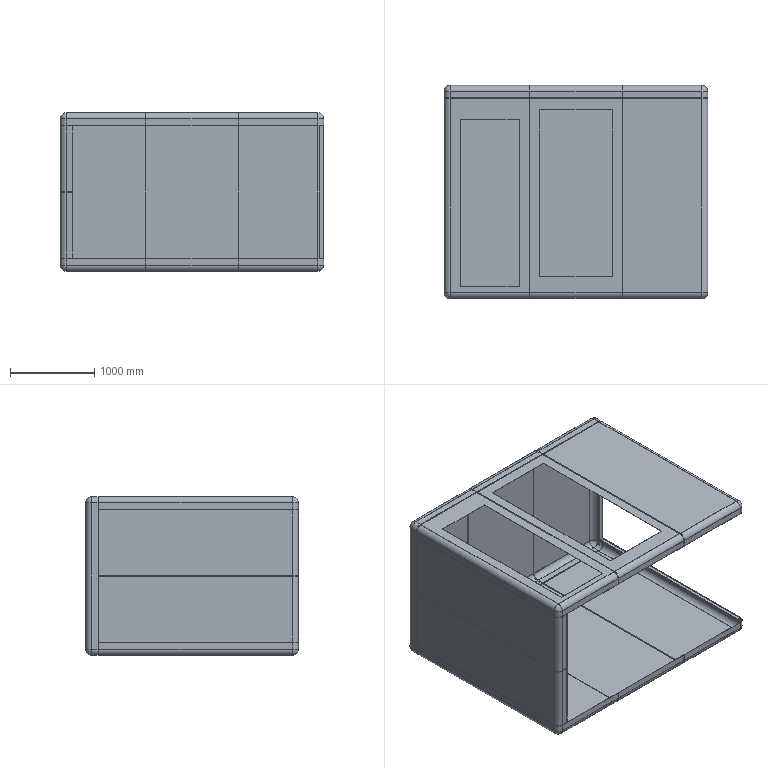Assembly | SolidWorks | mm | 23 component files | 23 solids | 472 faces | box 3131 x 2531 x 1881 mm | volume 75496655 mm3 | plane 358 | cylinder 98 | torus 16 | commonest cylinder face diameters 139 x35 133 x35 141 x8 135 x8 10 x6 4 x6
Bill of materials:
A-SideAluminumCasing1 | 1 |  | Thin rectangular frame-like plate with a large central rectangular opening; one long edge turns down with a rounded bend, forming a short flange.
A-SideAluminumCasing2 | 1 |  | Thin rectangular frame-like plate with a large central rectangular opening and one long edge rolled down into a short rounded flange.
A-SideAluminumCasing3 | 1 |  | Solid rectangular plate or shallow cover with no openings and rounded edges and corners on at least two adjacent sides.
A-SideSealant | 1 |  | Very thin, long sheet or strip; both ends appear turned through small rounded bends.
C-SideSealant1 | 7 |  | Very thin, long sheet or strip with a small rounded bend at one end only.
C-SideAluminumCasing1 | 1 |  | Flat rectangular sheet with one long edge bent down into a short flange with a small radius.
C-SideAluminumCasing2 | 1 |  | Rectangular sheet panel; one long edge is bent down and the opposite long edge appears turned up with a radius, giving an offset or stepped edge profile.
C-SideAluminumCasing3 | 1 |  | Rectangular tray-like sheet panel with a rounded downturned edge along one long side and short raised lips at the short ends.
C-SideSealant | 1 |  | Very thin, long sheet or strip with both ends turned through small rounded bends, apparently in the opposite direction to the similar strip parts.
D-SideAluminumCasing | 2 |  | Rectangular sheet panel standing on edge, with a short return flange formed by a small rounded bend along one edge (an L-like profile).
D-SideSealant | 1 |  | Flat thin rectangular sheet or plate with no visible holes, bends or edge features.
CasingA | 1 |  | Rectangular plate or panel of noticeable thickness with rounded edges and corners on several sides, giving a soft-edged slab shape.
CasingB | 1 |  | Thin-walled shallow channel (C-profile) with constant cross-section: a wide flat web with a short flange along each long edge, joined by radiused bends; both ends open.
CasingC | 1 |  | Thin-walled channel of similar C-profile to unnamed part, but closed at one end by an end wall with rounded corners, making a shallow tray-like cap; the other end is open.
Sealant | 2 |  | Very thin, narrow C-shaped profile element: a long straight segment with short angled/curved returns at each end. It looks like a thin slice of a channel profile or a sheet-thin surface body.
Mates:
1. coincident | C-SideAluminumHousingAssembly-1/C-SideAluminumCasing2-1 face at (-946, 0, -3) dir (0, 0, -1) | TopHousingAssembly-1/CasingA-1 face at (-476, 2458.5, -3) dir (0, 0, -1)
2. coincident | C-SideAluminumHousingAssembly-1/C-SideAluminumCasing2-1 face at (-1015.5, 0, 0) dir (-1, 0, 0) | TopHousingAssembly-1/CasingA-1 face at (-1015.5, 2458.5, 937.5) dir (-1, 0, 0)
3. coincident | C-SideAluminumHousingAssembly-1/C-SideSealant-1 face at (-946, 2312, -3) dir (0, 1, 0) | TopHousingAssembly-1/CasingA-1 face at (-6, 2312, 1878) dir (0, -1, 0)
4. coincident | C-SideAluminumHousingAssembly-1/C-SideAluminumCasing2-1 face at (-1015.5, 0, 0) dir (-1, 0, 0) | D-SideAluminumHousingAssembly-1/D-SideAluminumCasing-2 face at (-1015.5, 0, 152.5) dir (-1, 0, 0)
5. coincident | C-SideAluminumHousingAssembly-1/C-SideAluminumCasing2-1 face at (-946, -69.5, 0) dir (0, -1, 0) | D-SideAluminumHousingAssembly-1/D-SideAluminumCasing-2 face at (-1012.5, -69.5, 152.5) dir (0, -1, 0)
6. coincident | C-SideAluminumHousingAssembly-1/C-SideAluminumCasing2-1 face at (-945, -69.5, 146.5) dir (0, 0, 1) | D-SideAluminumHousingAssembly-1/C-SideSealant1-2 face at (-1012.5, 0, 146.5) dir (0, 0, -1)
7. coincident | TopHousingAssembly-1/CasingA-1 face at (-476, 2458.5, 1878) dir (0, 0, 1) | A-SideAluminumCasingAssembly-1/A-SideAluminumCasing1-1 face at (-946, 0, 1878) dir (0, 0, 1)
8. coincident | D-SideAluminumHousingAssembly-1/D-SideAluminumCasing-1 face at (-1015.5, 0, 940.5) dir (-1, 0, 0) | A-SideAluminumCasingAssembly-1/A-SideAluminumCasing1-1 face at (-1015.5, 0, 1875) dir (-1, 0, 0)
9. coincident | TopHousingAssembly-1/CasingA-1 face at (-6, 2312, 1878) dir (0, -1, 0) | A-SideAluminumCasingAssembly-1/A-SideSealant-1 face at (-946, 2312, 1878) dir (0, 1, 0)
10. coincident | A-SideAluminumCasingAssembly face at (0, 0, 0) dir (-1, 0, 0) | C-SideSealant1-1 face at (0, 0, 0) dir (1, 0, 0)
11. coincident | A-SideAluminumCasingAssembly face at (0, 0, 0) dir (0, 0, 1) | C-SideSealant1-1 face at (-3, 0, 0) dir (0, 0, 1)
12. coincident | A-SideAluminumCasingAssembly face at (0, -66.5, 0) dir (0, 1, 0) | C-SideSealant1-1 face at (-3, -66.5, 0) dir (0, 1, 0)
13. coincident | A-SideAluminumCasingAssembly face at (0, 0, 0) dir (0, 0, 1) | A-SideAluminumCasingAssembly face at (-946, 0, 0) dir (0, 0, 1)
14. coincident | A-SideAluminumCasingAssembly face at (0, -66.5, 0) dir (0, 1, 0) | A-SideAluminumCasingAssembly face at (-946, -66.5, 0) dir (0, 1, 0)
15. coincident | A-SideAluminumCasingAssembly face at (-6, 0, 0) dir (1, 0, 0) | C-SideSealant1-1 face at (-6, 0, 0) dir (-1, 0, 0)
16. coincident | A-SideAluminumCasingAssembly face at (0, 0, 0) dir (0, 0, 1) | A-SideAluminumCasing1-1 face at (2046, 0, 0) dir (0, 0, 1)
17. coincident | A-SideAluminumCasingAssembly face at (0, -66.5, 0) dir (0, 1, 0) | A-SideAluminumCasing1-1 face at (2046, -66.5, 0) dir (0, 1, 0)
18. coincident | A-SideAluminumCasingAssembly face at (0, 0, 0) dir (0, 0, 1) | A-SideAluminumCasing3-1 face at (-946, 0, 0) dir (0, 0, 1)
19. coincident | A-SideAluminumCasingAssembly face at (0, -66.5, 0) dir (0, 1, 0) | A-SideAluminumCasing3-1 face at (-946, -66.5, 0) dir (0, 1, 0)
20. coincident | C-SideSealant1-1 face at (-6, 0, 0) dir (-1, 0, 0) | A-SideAluminumCasing3-1 face at (-6, 0, 0) dir (1, 0, 0)
21. coincident | A-SideAluminumCasingAssembly face at (0, 2306, 0) dir (0, 1, 0) | A-SideSealant-1 face at (2046, 2306, -3) dir (0, -1, 0)
22. coincident | A-SideAluminumCasingAssembly face at (0, 0, 0) dir (0, 0, 1) | A-SideSealant-1 face at (2046, 2306, 0) dir (0, 0, 1)
23. coincident | A-SideAluminumCasing1-1 face at (2115.5, 0, 0) dir (1, 0, 0) | A-SideSealant-1 face at (2115.5, 2306, 0) dir (1, 0, 0)
24. coincident | A-SideAluminumCasing2-2 face at (0, 0, -3) dir (0, 0, -1) | A-SideAluminumCasing1-1 face at (2046, 0, -3) dir (0, 0, -1)
25. coincident | A-SideAluminumCasing2-2 face at (0, 2306, 0) dir (0, 1, 0) | A-SideSealant-1 face at (2046, 2306, -3) dir (0, -1, 0)
26. coincident | A-SideAluminumCasing2-2 face at (0, 0, 0) dir (0, 0, 1) | A-SideSealant-1 face at (2046, 2306, 0) dir (0, 0, 1)
27. coincident | A-SideAluminumCasing2-2 face at (0, 0, 0) dir (-1, 0, 0) | C-SideSealant1-1 face at (0, 0, 0) dir (1, 0, 0)
28. coincident | A-SideAluminumCasing2-2 face at (0, 0, -3) dir (0, 0, -1) | A-SideAluminumCasing3-1 face at (-946, 0, -3) dir (0, 0, -1)
29. coincident | A-SideAluminumCasing2-2 face at (0, -66.5, 0) dir (0, 1, 0) | A-SideAluminumCasing3-1 face at (-946, -66.5, 0) dir (0, 1, 0)
30. coincident | A-SideAluminumCasing2-2 face at (0, -66.5, 0) dir (0, 1, 0) | A-SideAluminumCasing1-1 face at (2046, -66.5, 0) dir (0, 1, 0)
31. coincident | A-SideAluminumCasing2-2 face at (0, 0, 0) dir (0, 0, 1) | C-SideSealant1-1 face at (-3, 0, 0) dir (0, 0, 1)
32. coincident | A-SideAluminumCasing2-2 face at (0, -66.5, 0) dir (0, 1, 0) | C-SideSealant1-1 face at (-3, -66.5, 0) dir (0, 1, 0)
33. coincident | A-SideAluminumCasing2-2 face at (0, 0, 0) dir (0, 0, 1) | C-SideSealant1-2 face at (1103, 0, 0) dir (0, 0, 1)
34. coincident | A-SideAluminumCasing2-2 face at (0, -66.5, 0) dir (0, 1, 0) | C-SideSealant1-2 face at (1103, -66.5, 0) dir (0, 1, 0)
35. coincident | A-SideAluminumCasing2-2 face at (1100, 0, 0) dir (1, 0, 0) | C-SideSealant1-2 face at (1100, 0, 0) dir (-1, 0, 0)
36. coincident | C-SideSealant1-2 face at (1106, 0, 0) dir (1, 0, 0) | A-SideAluminumCasing1-1 face at (1106, 0, 0) dir (-1, 0, 0)
37. coincident | C-SideAluminumCasing1-1 face at (0, 0, 0) dir (-1, 0, 0) | C-SideSealant1-1 face at (0, 0, 0) dir (1, 0, 0)
38. coincident | C-SideAluminumCasing1-1 face at (0, 0, 0) dir (0, 0, 1) | C-SideSealant1-1 face at (-3, 0, 0) dir (0, 0, 1)
39. coincident | C-SideAluminumCasing1-1 face at (0, -66.5, 0) dir (0, 1, 0) | C-SideSealant1-1 face at (-3, -66.5, 0) dir (0, 1, 0)
40. coincident | C-SideAluminumCasing1-1 face at (0, -66.5, 0) dir (0, 1, 0) | C-SideSealant1-2 face at (1103, -66.5, 0) dir (0, 1, 0)
41. coincident | C-SideAluminumCasing1-1 face at (0, 0, 0) dir (0, 0, 1) | C-SideSealant1-2 face at (1103, 0, 0) dir (0, 0, 1)
42. coincident | C-SideAluminumCasing1-1 face at (1100, 0, 0) dir (1, 0, 0) | C-SideSealant1-2 face at (1100, 0, 0) dir (-1, 0, 0)
43. coincident | C-SideAluminumCasing1-1 face at (0, 0, 0) dir (0, 0, 1) | C-SideAluminumCasing3-1 face at (2046, 0, 0) dir (0, 0, 1)
44. coincident | C-SideAluminumCasing1-1 face at (0, -66.5, 0) dir (0, 1, 0) | C-SideAluminumCasing3-1 face at (2046, -66.5, 0) dir (0, 1, 0)
45. coincident | C-SideAluminumCasing3-1 face at (1106, 0, 0) dir (-1, 0, 0) | C-SideSealant1-2 face at (1106, 0, 0) dir (1, 0, 0)
46. coincident | C-SideAluminumCasing1-1 face at (0, -66.5, 0) dir (0, 1, 0) | C-SideAluminumCasing2-1 face at (-946, -66.5, 0) dir (0, 1, 0)
47. coincident | C-SideAluminumCasing1-1 face at (0, 0, 0) dir (0, 0, 1) | C-SideAluminumCasing2-1 face at (-946, 0, 0) dir (0, 0, 1)
48. coincident | C-SideAluminumCasing2-1 face at (-6, 0, 0) dir (1, 0, 0) | C-SideSealant1-1 face at (-6, 0, 0) dir (-1, 0, 0)
49. coincident | C-SideAluminumCasing1-1 face at (0, 2306, 0) dir (0, 1, 0) | C-SideSealant-1 face at (-946, 2306, -3) dir (0, -1, 0)
50. coincident | C-SideAluminumCasing1-1 face at (0, 0, 0) dir (0, 0, 1) | C-SideSealant-1 face at (-946, 2312, 0) dir (0, 0, 1)
51. coincident | C-SideAluminumCasing2-1 face at (-1015.5, 0, 0) dir (-1, 0, 0) | C-SideSealant-1 face at (-1015.5, 2312, 0) dir (-1, 0, 0)
52. coincident | D-SideAluminumCasing-1 face at (0, 0, 0) dir (0, 0, -1) | D-SideAluminumCasing-2 face at (-788, 0, 0) dir (0, 0, -1)
53. coincident | D-SideAluminumCasing-1 face at (0, -66.5, 0) dir (0, 1, 0) | D-SideAluminumCasing-2 face at (-788, -66.5, 0) dir (0, 1, 0)
54. coincident | D-SideAluminumCasing-1 face at (0, -66.5, 0) dir (0, 1, 0) | C-SideSealant1-1 face at (-3, -66.5, 0) dir (0, 1, 0)
55. coincident | D-SideAluminumCasing-1 face at (0, 0, 3) dir (-1, 0, 0) | C-SideSealant1-1 face at (0, 0, 0) dir (1, 0, 0)
56. coincident | D-SideAluminumCasing-1 face at (0, 0, 0) dir (0, 0, -1) | C-SideSealant1-1 face at (-3, 0, 0) dir (0, 0, -1)
57. coincident | D-SideAluminumCasing-2 face at (-6, 0, 3) dir (1, 0, 0) | C-SideSealant1-1 face at (-6, 0, 0) dir (-1, 0, 0)
58. coincident | D-SideAluminumCasing-2 face at (-788, -66.5, 0) dir (0, 1, 0) | C-SideSealant1-2 face at (-791, -66.5, 0) dir (0, 1, 0)
59. coincident | D-SideAluminumCasing-2 face at (-788, 0, 0) dir (0, 0, -1) | C-SideSealant1-2 face at (-791, 0, 0) dir (0, 0, -1)
60. coincident | D-SideAluminumCasing-2 face at (-788, 0, 3) dir (-1, 0, 0) | C-SideSealant1-2 face at (-788, 0, 0) dir (1, 0, 0)
61. coincident | D-SideAluminumCasing-1 face at (0, -66.5, 0) dir (0, 1, 0) | C-SideSealant1-3 face at (785, -66.5, 0) dir (0, 1, 0)
62. coincident | D-SideAluminumCasing-1 face at (0, 0, 0) dir (0, 0, -1) | C-SideSealant1-3 face at (785, 0, 0) dir (0, 0, -1)
63. coincident | D-SideAluminumCasing-1 face at (782, 0, 3) dir (1, 0, 0) | C-SideSealant1-3 face at (782, 0, 0) dir (-1, 0, 0)
64. coincident | D-SideAluminumCasing-2 face at (-788, 0, 3) dir (0, 0, 1) | D-SideSealant-1 face at (-794, 2312, 3) dir (0, 0, 1)
65. coincident | D-SideAluminumCasing-2 face at (-788, 2306, 3) dir (0, 1, 0) | D-SideSealant-1 face at (-794, 2306, 3) dir (0, -1, 0)
66. coincident | C-SideSealant1-2 face at (-794, 0, 0) dir (-1, 0, 0) | D-SideSealant-1 face at (-794, 2306, 3) dir (-1, 0, 0)
67. coincident | CasingA-1 face at (470, 3, 871) dir (1, 0, 0) | Sealant-1 face at (470, 3, 871) dir (-1, 0, 0)
68. coincident | CasingA-1 face at (0, 0, 940.5) dir (0, 0, 1) | Sealant-1 face at (473, 0, 940.5) dir (0, 0, 1)
69. coincident | CasingA-1 face at (0, 3, 0) dir (0, 1, 0) | Sealant-1 face at (473, 3, 0) dir (0, 1, 0)
70. coincident | Sealant-1 face at (476, 3, 871) dir (1, 0, 0) | CasingB-1 face at (476, 3, 871) dir (-1, 0, 0)
71. coincident | CasingA-1 face at (0, 3, 0) dir (0, 1, 0) | CasingB-1 face at (1026, 3, 0) dir (0, 1, 0)
72. coincident | CasingA-1 face at (0, 0, 940.5) dir (0, 0, 1) | CasingB-1 face at (1026, 0, 940.5) dir (0, 0, 1)
73. coincident | CasingB-1 face at (1026, 3, 0) dir (0, 1, 0) | TopHousingAssembly face at (2052, 3, 0) dir (0, 1, 0)
74. coincident | CasingB-1 face at (1026, 0, 940.5) dir (0, 0, 1) | TopHousingAssembly face at (2052, 0, 940.5) dir (0, 0, 1)
75. coincident | CasingB-1 face at (1576, 3, 871) dir (1, 0, 0) | Sealant-2 face at (1576, 3, 871) dir (-1, 0, 0)
76. coincident | CasingB-1 face at (1026, 3, 0) dir (0, 1, 0) | Sealant-2 face at (1579, 3, 0) dir (0, 1, 0)
77. coincident | CasingB-1 face at (1026, 0, 940.5) dir (0, 0, 1) | Sealant-2 face at (1579, 0, 940.5) dir (0, 0, 1)
78. coincident | TopHousingAssembly face at (1582, 3, -871) dir (-1, 0, 0) | Sealant-2 face at (1582, 3, 871) dir (1, 0, 0)
79. coincident | CasingB-1 face at (1026, 0, 0) dir (0, -1, 0) | CasingC-1 face at (2052, 0, 0) dir (0, -1, 0)
80. coincident | CasingB-1 face at (1026, 0, 940.5) dir (0, 0, 1) | CasingC-1 face at (2052, 0, 940.5) dir (0, 0, 1)
81. coincident | Sealant-2 face at (1582, 3, 871) dir (1, 0, 0) | CasingC-1 face at (1582, 3, -871) dir (-1, 0, 0)